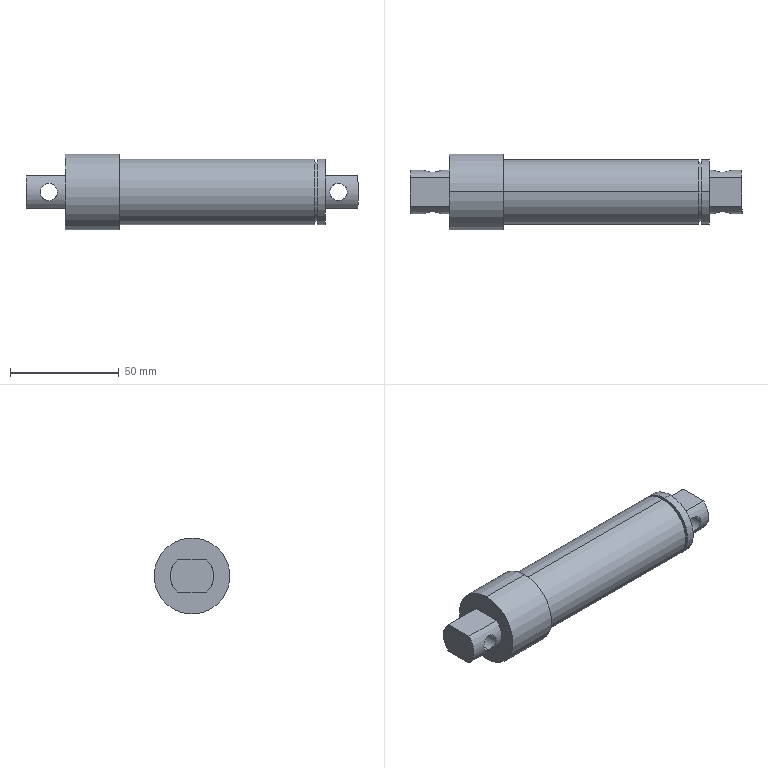Component | SolidWorks | LowerSideBeltXG-XG1-1_DrivenPulleyShaftXG-XG1-1 | 1 solid | 27 faces | box 153 x 35 x 35 mm | volume 97945 mm3 | cylinder 16 | plane 11 | commonest cylinder face diameters 8 x4 30 x4 20 x4 35 x2 27 x2
STEP:
#1=COLOUR_RGB('',0.7922,0.8196,0.9333);
#2=FILL_AREA_STYLE_COLOUR('',#1);
#3=FILL_AREA_STYLE('',(#2));
#4=SURFACE_STYLE_FILL_AREA(#3);
#5=SURFACE_SIDE_STYLE('',(#4));
#6=SURFACE_STYLE_USAGE(.BOTH.,#5);
#7=PRESENTATION_STYLE_ASSIGNMENT((#6));
#8=CARTESIAN_POINT('',(-7.489,10.853,4.331));
#9=VERTEX_POINT('',#8);
#10=CARTESIAN_POINT('',(-7.489,10.853,4.646));
#11=VERTEX_POINT('',#10);
#12=CARTESIAN_POINT('',(-7.489,10.853,4.331));
#13=CARTESIAN_POINT('',(-7.479,10.853,4.331));
#14=CARTESIAN_POINT('',(-7.468,10.853,4.332));
#15=CARTESIAN_POINT('',(-7.448,10.855,4.336));
#16=CARTESIAN_POINT('',(-7.438,10.856,4.339));
#17=CARTESIAN_POINT('',(-7.419,10.86,4.347));
#18=CARTESIAN_POINT('',(-7.41,10.861,4.352));
#19=CARTESIAN_POINT('',(-7.393,10.865,4.363));
#20=CARTESIAN_POINT('',(-7.385,10.868,4.37));
#21=CARTESIAN_POINT('',(-7.37,10.872,4.384));
#22=CARTESIAN_POINT('',(-7.364,10.874,4.392));
#23=CARTESIAN_POINT('',(-7.353,10.878,4.409));
#24=CARTESIAN_POINT('',(-7.348,10.88,4.418));
#25=CARTESIAN_POINT('',(-7.34,10.883,4.437));
#26=CARTESIAN_POINT('',(-7.337,10.884,4.447));
#27=CARTESIAN_POINT('',(-7.333,10.885,4.467));
#28=CARTESIAN_POINT('',(-7.331,10.886,4.478));
#29=CARTESIAN_POINT('',(-7.331,10.886,4.498));
#30=CARTESIAN_POINT('',(-7.332,10.885,4.509));
#31=CARTESIAN_POINT('',(-7.337,10.884,4.529));
#32=CARTESIAN_POINT('',(-7.34,10.883,4.539));
#33=CARTESIAN_POINT('',(-7.348,10.88,4.558));
#34=CARTESIAN_POINT('',(-7.352,10.878,4.567));
#35=CARTESIAN_POINT('',(-7.364,10.874,4.584));
#36=CARTESIAN_POINT('',(-7.37,10.872,4.592));
#37=CARTESIAN_POINT('',(-7.385,10.868,4.607));
#38=CARTESIAN_POINT('',(-7.393,10.865,4.613));
#39=CARTESIAN_POINT('',(-7.41,10.861,4.625));
#40=CARTESIAN_POINT('',(-7.419,10.86,4.629));
#41=CARTESIAN_POINT('',(-7.438,10.856,4.637));
#42=CARTESIAN_POINT('',(-7.448,10.855,4.641));
#43=CARTESIAN_POINT('',(-7.468,10.853,4.645));
#44=CARTESIAN_POINT('',(-7.478,10.853,4.646));
#45=CARTESIAN_POINT('',(-7.489,10.853,4.646));
#46=B_SPLINE_CURVE_WITH_KNOTS('',3,(#12,#13,#14,#15,#16,#17,#18,#19,#20,#21,#22,#23,#24,#25,#26,#27,#28,#29,#30,#31,#32,#33,#34,#35,#36,#37,#38,#39,#40,#41,#42,#43,#44,#45),.UNSPECIFIED.,.F.,.F.,(4,2,2,2,2,2,2,2,2,2,2,2,2,2,2,2,4),(0.01264,0.01343,0.01422,0.01501,0.0158,0.01658,0.01737,0.01816,0.01895,0.01974,0.02053,0.02132,0.02211,0.0229,0.02369,0.02448,0.02527),.UNSPECIFIED.);
#47=EDGE_CURVE('',#9,#11,#46,.T.);
#48=ORIENTED_EDGE('',*,*,#47,.F.);
#49=CARTESIAN_POINT('',(-7.489,10.131,4.331));
#50=VERTEX_POINT('',#49);
#51=CARTESIAN_POINT('',(-7.489,10.098,4.331));
#52=DIRECTION('',(0.,-1.,-0.));
#53=VECTOR('',#52,39.37);
#54=LINE('',#51,#53);
#55=EDGE_CURVE('',#9,#50,#54,.T.);
#56=ORIENTED_EDGE('',*,*,#55,.T.);
#57=CARTESIAN_POINT('',(-7.489,10.131,4.646));
#58=VERTEX_POINT('',#57);
#59=CARTESIAN_POINT('',(-7.489,10.131,4.646));
#60=CARTESIAN_POINT('',(-7.478,10.131,4.646));
#61=CARTESIAN_POINT('',(-7.468,10.131,4.645));
#62=CARTESIAN_POINT('',(-7.448,10.129,4.641));
#63=CARTESIAN_POINT('',(-7.438,10.128,4.637));
#64=CARTESIAN_POINT('',(-7.419,10.125,4.63));
#65=CARTESIAN_POINT('',(-7.41,10.123,4.625));
#66=CARTESIAN_POINT('',(-7.393,10.119,4.613));
#67=CARTESIAN_POINT('',(-7.385,10.117,4.607));
#68=CARTESIAN_POINT('',(-7.37,10.112,4.592));
#69=CARTESIAN_POINT('',(-7.364,10.11,4.584));
#70=CARTESIAN_POINT('',(-7.352,10.106,4.567));
#71=CARTESIAN_POINT('',(-7.348,10.105,4.558));
#72=CARTESIAN_POINT('',(-7.34,10.102,4.539));
#73=CARTESIAN_POINT('',(-7.337,10.1,4.529));
#74=CARTESIAN_POINT('',(-7.333,10.099,4.509));
#75=CARTESIAN_POINT('',(-7.331,10.098,4.499));
#76=CARTESIAN_POINT('',(-7.331,10.098,4.478));
#77=CARTESIAN_POINT('',(-7.333,10.099,4.467));
#78=CARTESIAN_POINT('',(-7.337,10.1,4.447));
#79=CARTESIAN_POINT('',(-7.34,10.102,4.437));
#80=CARTESIAN_POINT('',(-7.348,10.105,4.418));
#81=CARTESIAN_POINT('',(-7.353,10.106,4.409));
#82=CARTESIAN_POINT('',(-7.364,10.11,4.392));
#83=CARTESIAN_POINT('',(-7.371,10.112,4.384));
#84=CARTESIAN_POINT('',(-7.385,10.117,4.37));
#85=CARTESIAN_POINT('',(-7.393,10.119,4.363));
#86=CARTESIAN_POINT('',(-7.41,10.123,4.352));
#87=CARTESIAN_POINT('',(-7.419,10.125,4.347));
#88=CARTESIAN_POINT('',(-7.438,10.128,4.339));
#89=CARTESIAN_POINT('',(-7.448,10.129,4.336));
#90=CARTESIAN_POINT('',(-7.468,10.131,4.332));
#91=CARTESIAN_POINT('',(-7.479,10.131,4.331));
#92=CARTESIAN_POINT('',(-7.489,10.131,4.331));
#93=B_SPLINE_CURVE_WITH_KNOTS('',3,(#59,#60,#61,#62,#63,#64,#65,#66,#67,#68,#69,#70,#71,#72,#73,#74,#75,#76,#77,#78,#79,#80,#81,#82,#83,#84,#85,#86,#87,#88,#89,#90,#91,#92),.UNSPECIFIED.,.F.,.F.,(4,2,2,2,2,2,2,2,2,2,2,2,2,2,2,2,4),(0.,0.0007899,0.00158,0.00237,0.00316,0.00395,0.00474,0.00553,0.006319,0.007109,0.007899,0.008689,0.009479,0.01027,0.01106,0.01185,0.01264),.UNSPECIFIED.);
#94=EDGE_CURVE('',#58,#50,#93,.T.);
#95=ORIENTED_EDGE('',*,*,#94,.F.);
#96=CARTESIAN_POINT('',(-7.489,10.098,4.646));
#97=DIRECTION('',(0.,-1.,-0.));
#98=VECTOR('',#97,39.37);
#99=LINE('',#96,#98);
#100=EDGE_CURVE('',#11,#58,#99,.T.);
#101=ORIENTED_EDGE('',*,*,#100,.F.);
#102=EDGE_LOOP('',(#48,#56,#95,#101));
#103=FACE_OUTER_BOUND('',#102,.T.);
#104=CARTESIAN_POINT('',(-7.489,10.098,4.488));
#105=DIRECTION('',(0.,-1.,-0.));
#106=DIRECTION('',(0.,0.,1.));
#107=AXIS2_PLACEMENT_3D('',#104,#105,#106);
#108=CYLINDRICAL_SURFACE('',#107,0.1575);
#109=ADVANCED_FACE('',(#103),#108,.F.);
#110=CARTESIAN_POINT('',(-12.745,10.853,4.646));
#111=VERTEX_POINT('',#110);
#112=CARTESIAN_POINT('',(-12.745,10.853,4.331));
#113=VERTEX_POINT('',#112);
#114=CARTESIAN_POINT('',(-12.745,10.853,4.646));
#115=CARTESIAN_POINT('',(-12.734,10.853,4.646));
#116=CARTESIAN_POINT('',(-12.724,10.853,4.645));
#117=CARTESIAN_POINT('',(-12.704,10.855,4.641));
#118=CARTESIAN_POINT('',(-12.694,10.856,4.637));
#119=CARTESIAN_POINT('',(-12.675,10.86,4.63));
#120=CARTESIAN_POINT('',(-12.666,10.861,4.625));
#121=CARTESIAN_POINT('',(-12.649,10.865,4.613));
#122=CARTESIAN_POINT('',(-12.641,10.868,4.607));
#123=CARTESIAN_POINT('',(-12.626,10.872,4.592));
#124=CARTESIAN_POINT('',(-12.62,10.874,4.584));
#125=CARTESIAN_POINT('',(-12.608,10.878,4.567));
#126=CARTESIAN_POINT('',(-12.604,10.88,4.558));
#127=CARTESIAN_POINT('',(-12.596,10.883,4.539));
#128=CARTESIAN_POINT('',(-12.593,10.884,4.529));
#129=CARTESIAN_POINT('',(-12.588,10.885,4.509));
#130=CARTESIAN_POINT('',(-12.587,10.886,4.499));
#131=CARTESIAN_POINT('',(-12.587,10.886,4.478));
#132=CARTESIAN_POINT('',(-12.588,10.885,4.467));
#133=CARTESIAN_POINT('',(-12.593,10.884,4.447));
#134=CARTESIAN_POINT('',(-12.596,10.883,4.437));
#135=CARTESIAN_POINT('',(-12.604,10.88,4.418));
#136=CARTESIAN_POINT('',(-12.608,10.878,4.409));
#137=CARTESIAN_POINT('',(-12.62,10.874,4.392));
#138=CARTESIAN_POINT('',(-12.626,10.872,4.384));
#139=CARTESIAN_POINT('',(-12.641,10.868,4.37));
#140=CARTESIAN_POINT('',(-12.649,10.865,4.363));
#141=CARTESIAN_POINT('',(-12.666,10.861,4.352));
#142=CARTESIAN_POINT('',(-12.675,10.86,4.347));
#143=CARTESIAN_POINT('',(-12.694,10.856,4.339));
#144=CARTESIAN_POINT('',(-12.704,10.855,4.336));
#145=CARTESIAN_POINT('',(-12.724,10.853,4.332));
#146=CARTESIAN_POINT('',(-12.735,10.853,4.331));
#147=CARTESIAN_POINT('',(-12.745,10.853,4.331));
#148=B_SPLINE_CURVE_WITH_KNOTS('',3,(#114,#115,#116,#117,#118,#119,#120,#121,#122,#123,#124,#125,#126,#127,#128,#129,#130,#131,#132,#133,#134,#135,#136,#137,#138,#139,#140,#141,#142,#143,#144,#145,#146,#147),.UNSPECIFIED.,.F.,.F.,(4,2,2,2,2,2,2,2,2,2,2,2,2,2,2,2,4),(0.,0.0007899,0.00158,0.00237,0.00316,0.00395,0.00474,0.00553,0.006319,0.007109,0.007899,0.008689,0.009479,0.01027,0.01106,0.01185,0.01264),.UNSPECIFIED.);
#149=EDGE_CURVE('',#111,#113,#148,.T.);
#150=ORIENTED_EDGE('',*,*,#149,.T.);
#151=CARTESIAN_POINT('',(-12.745,10.131,4.331));
#152=VERTEX_POINT('',#151);
#153=CARTESIAN_POINT('',(-12.745,10.098,4.331));
#154=DIRECTION('',(0.,-1.,-0.));
#155=VECTOR('',#154,39.37);
#156=LINE('',#153,#155);
#157=EDGE_CURVE('',#113,#152,#156,.T.);
#158=ORIENTED_EDGE('',*,*,#157,.T.);
#159=CARTESIAN_POINT('',(-12.745,10.131,4.646));
#160=VERTEX_POINT('',#159);
#161=CARTESIAN_POINT('',(-12.745,10.131,4.331));
#162=CARTESIAN_POINT('',(-12.735,10.131,4.331));
#163=CARTESIAN_POINT('',(-12.724,10.131,4.332));
#164=CARTESIAN_POINT('',(-12.704,10.129,4.336));
#165=CARTESIAN_POINT('',(-12.694,10.128,4.339));
#166=CARTESIAN_POINT('',(-12.675,10.125,4.347));
#167=CARTESIAN_POINT('',(-12.666,10.123,4.352));
#168=CARTESIAN_POINT('',(-12.649,10.119,4.363));
#169=CARTESIAN_POINT('',(-12.641,10.117,4.37));
#170=CARTESIAN_POINT('',(-12.626,10.112,4.384));
#171=CARTESIAN_POINT('',(-12.62,10.11,4.392));
#172=CARTESIAN_POINT('',(-12.608,10.106,4.409));
#173=CARTESIAN_POINT('',(-12.604,10.105,4.418));
#174=CARTESIAN_POINT('',(-12.596,10.102,4.437));
#175=CARTESIAN_POINT('',(-12.593,10.1,4.447));
#176=CARTESIAN_POINT('',(-12.588,10.099,4.467));
#177=CARTESIAN_POINT('',(-12.587,10.098,4.478));
#178=CARTESIAN_POINT('',(-12.587,10.098,4.498));
#179=CARTESIAN_POINT('',(-12.588,10.099,4.509));
#180=CARTESIAN_POINT('',(-12.593,10.1,4.529));
#181=CARTESIAN_POINT('',(-12.596,10.102,4.539));
#182=CARTESIAN_POINT('',(-12.603,10.105,4.558));
#183=CARTESIAN_POINT('',(-12.608,10.106,4.567));
#184=CARTESIAN_POINT('',(-12.62,10.11,4.584));
#185=CARTESIAN_POINT('',(-12.626,10.112,4.592));
#186=CARTESIAN_POINT('',(-12.641,10.117,4.607));
#187=CARTESIAN_POINT('',(-12.649,10.119,4.613));
#188=CARTESIAN_POINT('',(-12.666,10.123,4.625));
#189=CARTESIAN_POINT('',(-12.675,10.125,4.629));
#190=CARTESIAN_POINT('',(-12.694,10.128,4.637));
#191=CARTESIAN_POINT('',(-12.704,10.129,4.641));
#192=CARTESIAN_POINT('',(-12.724,10.131,4.645));
#193=CARTESIAN_POINT('',(-12.734,10.131,4.646));
#194=CARTESIAN_POINT('',(-12.745,10.131,4.646));
#195=B_SPLINE_CURVE_WITH_KNOTS('',3,(#161,#162,#163,#164,#165,#166,#167,#168,#169,#170,#171,#172,#173,#174,#175,#176,#177,#178,#179,#180,#181,#182,#183,#184,#185,#186,#187,#188,#189,#190,#191,#192,#193,#194),.UNSPECIFIED.,.F.,.F.,(4,2,2,2,2,2,2,2,2,2,2,2,2,2,2,2,4),(0.01264,0.01343,0.01422,0.01501,0.0158,0.01658,0.01737,0.01816,0.01895,0.01974,0.02053,0.02132,0.02211,0.0229,0.02369,0.02448,0.02527),.UNSPECIFIED.);
#196=EDGE_CURVE('',#152,#160,#195,.T.);
#197=ORIENTED_EDGE('',*,*,#196,.T.);
#198=CARTESIAN_POINT('',(-12.745,10.098,4.646));
#199=DIRECTION('',(0.,-1.,-0.));
#200=VECTOR('',#199,39.37);
#201=LINE('',#198,#200);
#202=EDGE_CURVE('',#111,#160,#201,.T.);
#203=ORIENTED_EDGE('',*,*,#202,.F.);
#204=EDGE_LOOP('',(#150,#158,#197,#203));
#205=FACE_OUTER_BOUND('',#204,.T.);
#206=CARTESIAN_POINT('',(-12.745,10.098,4.488));
#207=DIRECTION('',(0.,-1.,-0.));
#208=DIRECTION('',(0.,0.,1.));
#209=AXIS2_PLACEMENT_3D('',#206,#207,#208);
#210=CYLINDRICAL_SURFACE('',#209,0.1575);
#211=ADVANCED_FACE('',(#205),#210,.F.);
#212=CARTESIAN_POINT('',(-12.45,10.492,3.799));
#213=VERTEX_POINT('',#212);
#214=CARTESIAN_POINT('',(-12.45,10.492,5.177));
#215=VERTEX_POINT('',#214);
#216=CARTESIAN_POINT('',(-12.45,10.492,4.488));
#217=DIRECTION('',(1.,0.,0.));
#218=DIRECTION('',(0.,0.,-1.));
#219=AXIS2_PLACEMENT_3D('',#216,#217,#218);
#220=CIRCLE('',#219,0.689);
#221=EDGE_CURVE('',#213,#215,#220,.T.);
#222=ORIENTED_EDGE('',*,*,#221,.T.);
#223=CARTESIAN_POINT('',(-11.465,10.492,5.177));
#224=VERTEX_POINT('',#223);
#225=CARTESIAN_POINT('',(13.589,10.492,5.177));
#226=DIRECTION('',(1.,0.,0.));
#227=VECTOR('',#226,39.37);
#228=LINE('',#225,#227);
#229=EDGE_CURVE('',#215,#224,#228,.T.);
#230=ORIENTED_EDGE('',*,*,#229,.T.);
#231=CARTESIAN_POINT('',(-11.465,10.492,3.799));
#232=VERTEX_POINT('',#231);
#233=CARTESIAN_POINT('',(-11.465,10.492,4.488));
#234=DIRECTION('',(1.,0.,0.));
#235=DIRECTION('',(0.,0.,-1.));
#236=AXIS2_PLACEMENT_3D('',#233,#234,#235);
#237=CIRCLE('',#236,0.689);
#238=EDGE_CURVE('',#232,#224,#237,.T.);
#239=ORIENTED_EDGE('',*,*,#238,.F.);
#240=CARTESIAN_POINT('',(13.589,10.492,3.799));
#241=DIRECTION('',(1.,0.,0.));
#242=VECTOR('',#241,39.37);
#243=LINE('',#240,#242);
#244=EDGE_CURVE('',#213,#232,#243,.T.);
#245=ORIENTED_EDGE('',*,*,#244,.F.);
#246=EDGE_LOOP('',(#222,#230,#239,#245));
#247=FACE_OUTER_BOUND('',#246,.T.);
#248=CARTESIAN_POINT('',(13.589,10.492,4.488));
#249=DIRECTION('',(1.,0.,0.));
#250=DIRECTION('',(0.,0.,-1.));
#251=AXIS2_PLACEMENT_3D('',#248,#249,#250);
#252=CYLINDRICAL_SURFACE('',#251,0.689);
#253=ADVANCED_FACE('',(#247),#252,.T.);
#254=CARTESIAN_POINT('',(-11.465,10.492,3.898));
#255=VERTEX_POINT('',#254);
#256=CARTESIAN_POINT('',(-11.465,10.492,5.079));
#257=VERTEX_POINT('',#256);
#258=CARTESIAN_POINT('',(-11.465,10.492,4.488));
#259=DIRECTION('',(1.,0.,0.));
#260=DIRECTION('',(0.,0.,-1.));
#261=AXIS2_PLACEMENT_3D('',#258,#259,#260);
#262=CIRCLE('',#261,0.5906);
#263=EDGE_CURVE('',#255,#257,#262,.T.);
#264=ORIENTED_EDGE('',*,*,#263,.T.);
#265=CARTESIAN_POINT('',(-7.922,10.492,5.079));
#266=VERTEX_POINT('',#265);
#267=CARTESIAN_POINT('',(13.589,10.492,5.079));
#268=DIRECTION('',(1.,0.,0.));
#269=VECTOR('',#268,39.37);
#270=LINE('',#267,#269);
#271=EDGE_CURVE('',#257,#266,#270,.T.);
#272=ORIENTED_EDGE('',*,*,#271,.T.);
#273=CARTESIAN_POINT('',(-7.922,10.492,3.898));
#274=VERTEX_POINT('',#273);
#275=CARTESIAN_POINT('',(-7.922,10.492,4.488));
#276=DIRECTION('',(1.,0.,0.));
#277=DIRECTION('',(0.,0.,-1.));
#278=AXIS2_PLACEMENT_3D('',#275,#276,#277);
#279=CIRCLE('',#278,0.5906);
#280=EDGE_CURVE('',#274,#266,#279,.T.);
#281=ORIENTED_EDGE('',*,*,#280,.F.);
#282=CARTESIAN_POINT('',(13.589,10.492,3.898));
#283=DIRECTION('',(1.,0.,0.));
#284=VECTOR('',#283,39.37);
#285=LINE('',#282,#284);
#286=EDGE_CURVE('',#255,#274,#285,.T.);
#287=ORIENTED_EDGE('',*,*,#286,.F.);
#288=EDGE_LOOP('',(#264,#272,#281,#287));
#289=FACE_OUTER_BOUND('',#288,.T.);
#290=CARTESIAN_POINT('',(13.589,10.492,4.488));
#291=DIRECTION('',(1.,0.,0.));
#292=DIRECTION('',(0.,0.,-1.));
#293=AXIS2_PLACEMENT_3D('',#290,#291,#292);
#294=CYLINDRICAL_SURFACE('',#293,0.5906);
#295=ADVANCED_FACE('',(#289),#294,.T.);
#296=CARTESIAN_POINT('',(-7.922,10.492,3.957));
#297=VERTEX_POINT('',#296);
#298=CARTESIAN_POINT('',(-7.922,10.492,5.02));
#299=VERTEX_POINT('',#298);
#300=CARTESIAN_POINT('',(-7.922,10.492,4.488));
#301=DIRECTION('',(1.,0.,0.));
#302=DIRECTION('',(0.,0.,-1.));
#303=AXIS2_PLACEMENT_3D('',#300,#301,#302);
#304=CIRCLE('',#303,0.5315);
#305=EDGE_CURVE('',#297,#299,#304,.T.);
#306=ORIENTED_EDGE('',*,*,#305,.T.);
#307=CARTESIAN_POINT('',(-7.875,10.492,5.02));
#308=VERTEX_POINT('',#307);
#309=CARTESIAN_POINT('',(13.589,10.492,5.02));
#310=DIRECTION('',(1.,0.,0.));
#311=VECTOR('',#310,39.37);
#312=LINE('',#309,#311);
#313=EDGE_CURVE('',#299,#308,#312,.T.);
#314=ORIENTED_EDGE('',*,*,#313,.T.);
#315=CARTESIAN_POINT('',(-7.875,10.492,3.957));
#316=VERTEX_POINT('',#315);
#317=CARTESIAN_POINT('',(-7.875,10.492,4.488));
#318=DIRECTION('',(1.,0.,0.));
#319=DIRECTION('',(0.,0.,-1.));
#320=AXIS2_PLACEMENT_3D('',#317,#318,#319);
#321=CIRCLE('',#320,0.5315);
#322=EDGE_CURVE('',#316,#308,#321,.T.);
#323=ORIENTED_EDGE('',*,*,#322,.F.);
#324=CARTESIAN_POINT('',(13.589,10.492,3.957));
#325=DIRECTION('',(1.,0.,0.));
#326=VECTOR('',#325,39.37);
#327=LINE('',#324,#326);
#328=EDGE_CURVE('',#297,#316,#327,.T.);
#329=ORIENTED_EDGE('',*,*,#328,.F.);
#330=EDGE_LOOP('',(#306,#314,#323,#329));
#331=FACE_OUTER_BOUND('',#330,.T.);
#332=CARTESIAN_POINT('',(13.589,10.492,4.488));
#333=DIRECTION('',(1.,0.,0.));
#334=DIRECTION('',(0.,0.,-1.));
#335=AXIS2_PLACEMENT_3D('',#332,#333,#334);
#336=CYLINDRICAL_SURFACE('',#335,0.5315);
#337=ADVANCED_FACE('',(#331),#336,.T.);
#338=CARTESIAN_POINT('',(-7.875,10.492,3.898));
#339=VERTEX_POINT('',#338);
#340=CARTESIAN_POINT('',(-7.875,10.492,5.079));
#341=VERTEX_POINT('',#340);
#342=CARTESIAN_POINT('',(-7.875,10.492,4.488));
#343=DIRECTION('',(1.,0.,0.));
#344=DIRECTION('',(0.,0.,-1.));
#345=AXIS2_PLACEMENT_3D('',#342,#343,#344);
#346=CIRCLE('',#345,0.5906);
#347=EDGE_CURVE('',#339,#341,#346,.T.);
#348=ORIENTED_EDGE('',*,*,#347,.T.);
#349=CARTESIAN_POINT('',(-7.725,10.492,5.079));
#350=VERTEX_POINT('',#349);
#351=CARTESIAN_POINT('',(13.589,10.492,5.079));
#352=DIRECTION('',(1.,0.,0.));
#353=VECTOR('',#352,39.37);
#354=LINE('',#351,#353);
#355=EDGE_CURVE('',#341,#350,#354,.T.);
#356=ORIENTED_EDGE('',*,*,#355,.T.);
#357=CARTESIAN_POINT('',(-7.725,10.492,3.898));
#358=VERTEX_POINT('',#357);
#359=CARTESIAN_POINT('',(-7.725,10.492,4.488));
#360=DIRECTION('',(1.,0.,0.));
#361=DIRECTION('',(0.,0.,-1.));
#362=AXIS2_PLACEMENT_3D('',#359,#360,#361);
#363=CIRCLE('',#362,0.5906);
#364=EDGE_CURVE('',#358,#350,#363,.T.);
#365=ORIENTED_EDGE('',*,*,#364,.F.);
#366=CARTESIAN_POINT('',(13.589,10.492,3.898));
#367=DIRECTION('',(1.,0.,0.));
#368=VECTOR('',#367,39.37);
#369=LINE('',#366,#368);
#370=EDGE_CURVE('',#339,#358,#369,.T.);
#371=ORIENTED_EDGE('',*,*,#370,.F.);
#372=EDGE_LOOP('',(#348,#356,#365,#371));
#373=FACE_OUTER_BOUND('',#372,.T.);
#374=CARTESIAN_POINT('',(13.589,10.492,4.488));
#375=DIRECTION('',(1.,0.,0.));
#376=DIRECTION('',(0.,0.,-1.));
#377=AXIS2_PLACEMENT_3D('',#374,#375,#376);
#378=CYLINDRICAL_SURFACE('',#377,0.5906);
#379=ADVANCED_FACE('',(#373),#378,.T.);
#380=CARTESIAN_POINT('',(-12.745,10.131,4.646));
#381=CARTESIAN_POINT('',(-12.755,10.131,4.646));
#382=CARTESIAN_POINT('',(-12.766,10.131,4.645));
#383=CARTESIAN_POINT('',(-12.786,10.129,4.641));
#384=CARTESIAN_POINT('',(-12.796,10.128,4.637));
#385=CARTESIAN_POINT('',(-12.815,10.125,4.63));
#386=CARTESIAN_POINT('',(-12.824,10.123,4.625));
#387=CARTESIAN_POINT('',(-12.841,10.119,4.613));
#388=CARTESIAN_POINT('',(-12.849,10.117,4.607));
#389=CARTESIAN_POINT('',(-12.863,10.112,4.592));
#390=CARTESIAN_POINT('',(-12.87,10.11,4.584));
#391=CARTESIAN_POINT('',(-12.881,10.106,4.567));
#392=CARTESIAN_POINT('',(-12.886,10.105,4.558));
#393=CARTESIAN_POINT('',(-12.894,10.102,4.539));
#394=CARTESIAN_POINT('',(-12.897,10.1,4.529));
#395=CARTESIAN_POINT('',(-12.901,10.099,4.509));
#396=CARTESIAN_POINT('',(-12.902,10.098,4.499));
#397=CARTESIAN_POINT('',(-12.902,10.098,4.478));
#398=CARTESIAN_POINT('',(-12.901,10.099,4.467));
#399=CARTESIAN_POINT('',(-12.897,10.1,4.447));
#400=CARTESIAN_POINT('',(-12.894,10.102,4.437));
#401=CARTESIAN_POINT('',(-12.886,10.105,4.418));
#402=CARTESIAN_POINT('',(-12.881,10.106,4.409));
#403=CARTESIAN_POINT('',(-12.87,10.11,4.392));
#404=CARTESIAN_POINT('',(-12.863,10.112,4.384));
#405=CARTESIAN_POINT('',(-12.849,10.117,4.37));
#406=CARTESIAN_POINT('',(-12.841,10.119,4.363));
#407=CARTESIAN_POINT('',(-12.824,10.123,4.352));
#408=CARTESIAN_POINT('',(-12.815,10.125,4.347));
#409=CARTESIAN_POINT('',(-12.796,10.128,4.339));
#410=CARTESIAN_POINT('',(-12.786,10.129,4.336));
#411=CARTESIAN_POINT('',(-12.766,10.131,4.332));
#412=CARTESIAN_POINT('',(-12.755,10.131,4.331));
#413=CARTESIAN_POINT('',(-12.745,10.131,4.331));
#414=B_SPLINE_CURVE_WITH_KNOTS('',3,(#380,#381,#382,#383,#384,#385,#386,#387,#388,#389,#390,#391,#392,#393,#394,#395,#396,#397,#398,#399,#400,#401,#402,#403,#404,#405,#406,#407,#408,#409,#410,#411,#412,#413),.UNSPECIFIED.,.F.,.F.,(4,2,2,2,2,2,2,2,2,2,2,2,2,2,2,2,4),(0.,0.0007899,0.00158,0.00237,0.00316,0.00395,0.00474,0.00553,0.006319,0.007109,0.007899,0.008689,0.009479,0.01027,0.01106,0.01185,0.01264),.UNSPECIFIED.);
#415=EDGE_CURVE('',#160,#152,#414,.T.);
#416=ORIENTED_EDGE('',*,*,#415,.F.);
#417=ORIENTED_EDGE('',*,*,#196,.F.);
#418=EDGE_LOOP('',(#416,#417));
#419=FACE_BOUND('',#418,.T.);
#420=CARTESIAN_POINT('',(-13.158,10.232,4.783));
#421=VERTEX_POINT('',#420);
#422=CARTESIAN_POINT('',(-12.45,10.232,4.783));
#423=VERTEX_POINT('',#422);
#424=CARTESIAN_POINT('',(-12.45,10.232,4.783));
#425=DIRECTION('',(1.,0.,0.));
#426=VECTOR('',#425,39.37);
#427=LINE('',#424,#426);
#428=EDGE_CURVE('',#421,#423,#427,.T.);
#429=ORIENTED_EDGE('',*,*,#428,.F.);
#430=CARTESIAN_POINT('',(-13.158,10.232,4.193));
#431=VERTEX_POINT('',#430);
#432=CARTESIAN_POINT('',(-13.158,10.492,4.488));
#433=DIRECTION('',(1.,0.,0.));
#434=DIRECTION('',(0.,0.,-1.));
#435=AXIS2_PLACEMENT_3D('',#432,#433,#434);
#436=CIRCLE('',#435,0.3937);
#437=EDGE_CURVE('',#421,#431,#436,.T.);
#438=ORIENTED_EDGE('',*,*,#437,.T.);
#439=CARTESIAN_POINT('',(-12.45,10.232,4.193));
#440=VERTEX_POINT('',#439);
#441=CARTESIAN_POINT('',(-12.45,10.232,4.193));
#442=DIRECTION('',(-1.,-0.,-0.));
#443=VECTOR('',#442,39.37);
#444=LINE('',#441,#443);
#445=EDGE_CURVE('',#440,#431,#444,.T.);
#446=ORIENTED_EDGE('',*,*,#445,.F.);
#447=CARTESIAN_POINT('',(-12.45,10.492,4.488));
#448=DIRECTION('',(-1.,-0.,-0.));
#449=DIRECTION('',(0.,0.,1.));
#450=AXIS2_PLACEMENT_3D('',#447,#448,#449);
#451=CIRCLE('',#450,0.3937);
#452=EDGE_CURVE('',#440,#423,#451,.T.);
#453=ORIENTED_EDGE('',*,*,#452,.T.);
#454=EDGE_LOOP('',(#429,#438,#446,#453));
#455=FACE_OUTER_BOUND('',#454,.T.);
#456=CARTESIAN_POINT('',(-12.45,10.492,4.488));
#457=DIRECTION('',(-1.,-0.,-0.));
#458=DIRECTION('',(0.,0.,1.));
#459=AXIS2_PLACEMENT_3D('',#456,#457,#458);
#460=CYLINDRICAL_SURFACE('',#459,0.3937);
#461=ADVANCED_FACE('',(#419,#455),#460,.T.);
#462=ORIENTED_EDGE('',*,*,#94,.T.);
#463=CARTESIAN_POINT('',(-7.489,10.131,4.331));
#464=CARTESIAN_POINT('',(-7.499,10.131,4.331));
#465=CARTESIAN_POINT('',(-7.51,10.131,4.332));
#466=CARTESIAN_POINT('',(-7.53,10.129,4.336));
#467=CARTESIAN_POINT('',(-7.54,10.128,4.339));
#468=CARTESIAN_POINT('',(-7.559,10.125,4.347));
#469=CARTESIAN_POINT('',(-7.568,10.123,4.352));
#470=CARTESIAN_POINT('',(-7.585,10.119,4.363));
#471=CARTESIAN_POINT('',(-7.593,10.117,4.37));
#472=CARTESIAN_POINT('',(-7.608,10.112,4.384));
#473=CARTESIAN_POINT('',(-7.614,10.11,4.392));
#474=CARTESIAN_POINT('',(-7.625,10.106,4.409));
#475=CARTESIAN_POINT('',(-7.63,10.105,4.418));
#476=CARTESIAN_POINT('',(-7.638,10.102,4.437));
#477=CARTESIAN_POINT('',(-7.641,10.1,4.447));
#478=CARTESIAN_POINT('',(-7.645,10.099,4.467));
#479=CARTESIAN_POINT('',(-7.646,10.098,4.478));
#480=CARTESIAN_POINT('',(-7.646,10.098,4.498));
#481=CARTESIAN_POINT('',(-7.645,10.099,4.509));
#482=CARTESIAN_POINT('',(-7.641,10.1,4.529));
#483=CARTESIAN_POINT('',(-7.638,10.102,4.539));
#484=CARTESIAN_POINT('',(-7.63,10.105,4.558));
#485=CARTESIAN_POINT('',(-7.625,10.106,4.567));
#486=CARTESIAN_POINT('',(-7.614,10.11,4.584));
#487=CARTESIAN_POINT('',(-7.608,10.112,4.592));
#488=CARTESIAN_POINT('',(-7.593,10.117,4.607));
#489=CARTESIAN_POINT('',(-7.585,10.119,4.613));
#490=CARTESIAN_POINT('',(-7.568,10.123,4.625));
#491=CARTESIAN_POINT('',(-7.559,10.125,4.629));
#492=CARTESIAN_POINT('',(-7.54,10.128,4.637));
#493=CARTESIAN_POINT('',(-7.53,10.129,4.641));
#494=CARTESIAN_POINT('',(-7.51,10.131,4.645));
#495=CARTESIAN_POINT('',(-7.499,10.131,4.646));
#496=CARTESIAN_POINT('',(-7.489,10.131,4.646));
#497=B_SPLINE_CURVE_WITH_KNOTS('',3,(#463,#464,#465,#466,#467,#468,#469,#470,#471,#472,#473,#474,#475,#476,#477,#478,#479,#480,#481,#482,#483,#484,#485,#486,#487,#488,#489,#490,#491,#492,#493,#494,#495,#496),.UNSPECIFIED.,.F.,.F.,(4,2,2,2,2,2,2,2,2,2,2,2,2,2,2,2,4),(0.01264,0.01343,0.01422,0.01501,0.0158,0.01658,0.01737,0.01816,0.01895,0.01974,0.02053,0.02132,0.02211,0.0229,0.02369,0.02448,0.02527),.UNSPECIFIED.);
#498=EDGE_CURVE('',#50,#58,#497,.T.);
#499=ORIENTED_EDGE('',*,*,#498,.T.);
#500=EDGE_LOOP('',(#462,#499));
#501=FACE_BOUND('',#500,.T.);
#502=CARTESIAN_POINT('',(-7.135,10.232,4.783));
#503=VERTEX_POINT('',#502);
#504=CARTESIAN_POINT('',(-7.135,10.232,4.193));
#505=VERTEX_POINT('',#504);
#506=CARTESIAN_POINT('',(-7.135,10.492,4.488));
#507=DIRECTION('',(1.,0.,0.));
#508=DIRECTION('',(0.,0.,-1.));
#509=AXIS2_PLACEMENT_3D('',#506,#507,#508);
#510=CIRCLE('',#509,0.3937);
#511=EDGE_CURVE('',#503,#505,#510,.T.);
#512=ORIENTED_EDGE('',*,*,#511,.F.);
#513=CARTESIAN_POINT('',(-7.725,10.232,4.783));
#514=VERTEX_POINT('',#513);
#515=CARTESIAN_POINT('',(13.589,10.232,4.783));
#516=DIRECTION('',(-1.,-0.,-0.));
#517=VECTOR('',#516,39.37);
#518=LINE('',#515,#517);
#519=EDGE_CURVE('',#503,#514,#518,.T.);
#520=ORIENTED_EDGE('',*,*,#519,.T.);
#521=CARTESIAN_POINT('',(-7.725,10.232,4.193));
#522=VERTEX_POINT('',#521);
#523=CARTESIAN_POINT('',(-7.725,10.492,4.488));
#524=DIRECTION('',(1.,0.,0.));
#525=DIRECTION('',(0.,0.,-1.));
#526=AXIS2_PLACEMENT_3D('',#523,#524,#525);
#527=CIRCLE('',#526,0.3937);
#528=EDGE_CURVE('',#514,#522,#527,.T.);
#529=ORIENTED_EDGE('',*,*,#528,.T.);
#530=CARTESIAN_POINT('',(13.589,10.232,4.193));
#531=DIRECTION('',(1.,0.,0.));
#532=VECTOR('',#531,39.37);
#533=LINE('',#530,#532);
#534=EDGE_CURVE('',#522,#505,#533,.T.);
#535=ORIENTED_EDGE('',*,*,#534,.T.);
#536=EDGE_LOOP('',(#512,#520,#529,#535));
#537=FACE_OUTER_BOUND('',#536,.T.);
#538=CARTESIAN_POINT('',(13.589,10.492,4.488));
#539=DIRECTION('',(1.,0.,0.));
#540=DIRECTION('',(0.,0.,-1.));
#541=AXIS2_PLACEMENT_3D('',#538,#539,#540);
#542=CYLINDRICAL_SURFACE('',#541,0.3937);
#543=ADVANCED_FACE('',(#501,#537),#542,.T.);
#544=CARTESIAN_POINT('',(-7.489,10.853,4.646));
#545=CARTESIAN_POINT('',(-7.499,10.853,4.646));
#546=CARTESIAN_POINT('',(-7.51,10.853,4.645));
#547=CARTESIAN_POINT('',(-7.53,10.855,4.641));
#548=CARTESIAN_POINT('',(-7.54,10.856,4.637));
#549=CARTESIAN_POINT('',(-7.559,10.86,4.63));
#550=CARTESIAN_POINT('',(-7.568,10.861,4.625));
#551=CARTESIAN_POINT('',(-7.585,10.865,4.613));
#552=CARTESIAN_POINT('',(-7.593,10.868,4.607));
#553=CARTESIAN_POINT('',(-7.608,10.872,4.592));
#554=CARTESIAN_POINT('',(-7.614,10.874,4.584));
#555=CARTESIAN_POINT('',(-7.626,10.878,4.567));
#556=CARTESIAN_POINT('',(-7.63,10.88,4.558));
#557=CARTESIAN_POINT('',(-7.638,10.883,4.539));
#558=CARTESIAN_POINT('',(-7.641,10.884,4.529));
#559=CARTESIAN_POINT('',(-7.645,10.885,4.509));
#560=CARTESIAN_POINT('',(-7.646,10.886,4.499));
#561=CARTESIAN_POINT('',(-7.646,10.886,4.478));
#562=CARTESIAN_POINT('',(-7.645,10.885,4.467));
#563=CARTESIAN_POINT('',(-7.641,10.884,4.447));
#564=CARTESIAN_POINT('',(-7.638,10.883,4.437));
#565=CARTESIAN_POINT('',(-7.63,10.88,4.418));
#566=CARTESIAN_POINT('',(-7.625,10.878,4.409));
#567=CARTESIAN_POINT('',(-7.614,10.874,4.392));
#568=CARTESIAN_POINT('',(-7.607,10.872,4.384));
#569=CARTESIAN_POINT('',(-7.593,10.868,4.37));
#570=CARTESIAN_POINT('',(-7.585,10.865,4.363));
#571=CARTESIAN_POINT('',(-7.568,10.861,4.352));
#572=CARTESIAN_POINT('',(-7.559,10.86,4.347));
#573=CARTESIAN_POINT('',(-7.54,10.856,4.339));
#574=CARTESIAN_POINT('',(-7.53,10.855,4.336));
#575=CARTESIAN_POINT('',(-7.51,10.853,4.332));
#576=CARTESIAN_POINT('',(-7.499,10.853,4.331));
#577=CARTESIAN_POINT('',(-7.489,10.853,4.331));
#578=B_SPLINE_CURVE_WITH_KNOTS('',3,(#544,#545,#546,#547,#548,#549,#550,#551,#552,#553,#554,#555,#556,#557,#558,#559,#560,#561,#562,#563,#564,#565,#566,#567,#568,#569,#570,#571,#572,#573,#574,#575,#576,#577),.UNSPECIFIED.,.F.,.F.,(4,2,2,2,2,2,2,2,2,2,2,2,2,2,2,2,4),(0.,0.0007899,0.00158,0.00237,0.00316,0.00395,0.00474,0.00553,0.006319,0.007109,0.007899,0.008689,0.009479,0.01027,0.01106,0.01185,0.01264),.UNSPECIFIED.);
#579=EDGE_CURVE('',#11,#9,#578,.T.);
#580=ORIENTED_EDGE('',*,*,#579,.T.);
#581=ORIENTED_EDGE('',*,*,#47,.T.);
#582=EDGE_LOOP('',(#580,#581));
#583=FACE_BOUND('',#582,.T.);
#584=CARTESIAN_POINT('',(-7.135,10.753,4.193));
#585=VERTEX_POINT('',#584);
#586=CARTESIAN_POINT('',(-7.135,10.753,4.783));
#587=VERTEX_POINT('',#586);
#588=CARTESIAN_POINT('',(-7.135,10.492,4.488));
#589=DIRECTION('',(1.,0.,0.));
#590=DIRECTION('',(0.,0.,-1.));
#591=AXIS2_PLACEMENT_3D('',#588,#589,#590);
#592=CIRCLE('',#591,0.3937);
#593=EDGE_CURVE('',#585,#587,#592,.T.);
#594=ORIENTED_EDGE('',*,*,#593,.F.);
#595=CARTESIAN_POINT('',(-7.725,10.753,4.193));
#596=VERTEX_POINT('',#595);
#597=CARTESIAN_POINT('',(13.589,10.753,4.193));
#598=DIRECTION('',(-1.,-0.,-0.));
#599=VECTOR('',#598,39.37);
#600=LINE('',#597,#599);
#601=EDGE_CURVE('',#585,#596,#600,.T.);
#602=ORIENTED_EDGE('',*,*,#601,.T.);
#603=CARTESIAN_POINT('',(-7.725,10.753,4.783));
#604=VERTEX_POINT('',#603);
#605=CARTESIAN_POINT('',(-7.725,10.492,4.488));
#606=DIRECTION('',(1.,0.,0.));
#607=DIRECTION('',(0.,0.,-1.));
#608=AXIS2_PLACEMENT_3D('',#605,#606,#607);
#609=CIRCLE('',#608,0.3937);
#610=EDGE_CURVE('',#596,#604,#609,.T.);
#611=ORIENTED_EDGE('',*,*,#610,.T.);
#612=CARTESIAN_POINT('',(13.589,10.753,4.783));
#613=DIRECTION('',(1.,0.,0.));
#614=VECTOR('',#613,39.37);
#615=LINE('',#612,#614);
#616=EDGE_CURVE('',#604,#587,#615,.T.);
#617=ORIENTED_EDGE('',*,*,#616,.T.);
#618=EDGE_LOOP('',(#594,#602,#611,#617));
#619=FACE_OUTER_BOUND('',#618,.T.);
#620=CARTESIAN_POINT('',(13.589,10.492,4.488));
#621=DIRECTION('',(1.,0.,0.));
#622=DIRECTION('',(0.,0.,-1.));
#623=AXIS2_PLACEMENT_3D('',#620,#621,#622);
#624=CYLINDRICAL_SURFACE('',#623,0.3937);
#625=ADVANCED_FACE('',(#583,#619),#624,.T.);
#626=CARTESIAN_POINT('',(-7.135,10.753,4.783));
#627=DIRECTION('',(0.,-1.,-0.));
#628=VECTOR('',#627,39.37);
#629=LINE('',#626,#628);
#630=EDGE_CURVE('',#587,#503,#629,.T.);
#631=ORIENTED_EDGE('',*,*,#630,.F.);
#632=ORIENTED_EDGE('',*,*,#616,.F.);
#633=CARTESIAN_POINT('',(-7.725,11.283,4.783));
#634=DIRECTION('',(-0.,1.,0.));
#635=VECTOR('',#634,39.37);
#636=LINE('',#633,#635);
#637=EDGE_CURVE('',#514,#604,#636,.T.);
#638=ORIENTED_EDGE('',*,*,#637,.F.);
#639=ORIENTED_EDGE('',*,*,#519,.F.);
#640=EDGE_LOOP('',(#631,#632,#638,#639));
#641=FACE_OUTER_BOUND('',#640,.T.);
#642=CARTESIAN_POINT('',(-7.725,11.283,4.783));
#643=DIRECTION('',(0.,0.,-1.));
#644=DIRECTION('',(0.,-1.,-0.));
#645=AXIS2_PLACEMENT_3D('',#642,#643,#644);
#646=PLANE('',#645);
#647=ADVANCED_FACE('',(#641),#646,.F.);
#648=CARTESIAN_POINT('',(-7.135,10.232,4.193));
#649=DIRECTION('',(-0.,1.,0.));
#650=VECTOR('',#649,39.37);
#651=LINE('',#648,#650);
#652=EDGE_CURVE('',#505,#585,#651,.T.);
#653=ORIENTED_EDGE('',*,*,#652,.F.);
#654=ORIENTED_EDGE('',*,*,#534,.F.);
#655=CARTESIAN_POINT('',(-7.725,11.283,4.193));
#656=DIRECTION('',(0.,-1.,-0.));
#657=VECTOR('',#656,39.37);
#658=LINE('',#655,#657);
#659=EDGE_CURVE('',#596,#522,#658,.T.);
#660=ORIENTED_EDGE('',*,*,#659,.F.);
#661=ORIENTED_EDGE('',*,*,#601,.F.);
#662=EDGE_LOOP('',(#653,#654,#660,#661));
#663=FACE_OUTER_BOUND('',#662,.T.);
#664=CARTESIAN_POINT('',(-7.725,11.283,4.193));
#665=DIRECTION('',(-0.,-0.,1.));
#666=DIRECTION('',(-0.,1.,0.));
#667=AXIS2_PLACEMENT_3D('',#664,#665,#666);
#668=PLANE('',#667);
#669=ADVANCED_FACE('',(#663),#668,.F.);
#670=ORIENTED_EDGE('',*,*,#610,.F.);
#671=ORIENTED_EDGE('',*,*,#659,.T.);
#672=ORIENTED_EDGE('',*,*,#528,.F.);
#673=ORIENTED_EDGE('',*,*,#637,.T.);
#674=EDGE_LOOP('',(#670,#671,#672,#673));
#675=FACE_BOUND('',#674,.T.);
#676=ORIENTED_EDGE('',*,*,#364,.T.);
#677=CARTESIAN_POINT('',(-7.725,10.492,4.488));
#678=DIRECTION('',(1.,0.,0.));
#679=DIRECTION('',(0.,0.,-1.));
#680=AXIS2_PLACEMENT_3D('',#677,#678,#679);
#681=CIRCLE('',#680,0.5906);
#682=EDGE_CURVE('',#350,#358,#681,.T.);
#683=ORIENTED_EDGE('',*,*,#682,.T.);
#684=EDGE_LOOP('',(#676,#683));
#685=FACE_OUTER_BOUND('',#684,.T.);
#686=CARTESIAN_POINT('',(-7.725,10.492,4.882));
#687=DIRECTION('',(-1.,-0.,-0.));
#688=DIRECTION('',(-0.,-0.,1.));
#689=AXIS2_PLACEMENT_3D('',#686,#687,#688);
#690=PLANE('',#689);
#691=ADVANCED_FACE('',(#675,#685),#690,.F.);
#692=ORIENTED_EDGE('',*,*,#355,.F.);
#693=CARTESIAN_POINT('',(-7.875,10.492,4.488));
#694=DIRECTION('',(1.,0.,0.));
#695=DIRECTION('',(0.,0.,-1.));
#696=AXIS2_PLACEMENT_3D('',#693,#694,#695);
#697=CIRCLE('',#696,0.5906);
#698=EDGE_CURVE('',#341,#339,#697,.T.);
#699=ORIENTED_EDGE('',*,*,#698,.T.);
#700=ORIENTED_EDGE('',*,*,#370,.T.);
#701=ORIENTED_EDGE('',*,*,#682,.F.);
#702=EDGE_LOOP('',(#692,#699,#700,#701));
#703=FACE_OUTER_BOUND('',#702,.T.);
#704=CARTESIAN_POINT('',(13.589,10.492,4.488));
#705=DIRECTION('',(1.,0.,0.));
#706=DIRECTION('',(0.,0.,-1.));
#707=AXIS2_PLACEMENT_3D('',#704,#705,#706);
#708=CYLINDRICAL_SURFACE('',#707,0.5906);
#709=ADVANCED_FACE('',(#703),#708,.T.);
#710=ORIENTED_EDGE('',*,*,#347,.F.);
#711=ORIENTED_EDGE('',*,*,#698,.F.);
#712=EDGE_LOOP('',(#710,#711));
#713=FACE_OUTER_BOUND('',#712,.T.);
#714=ORIENTED_EDGE('',*,*,#322,.T.);
#715=CARTESIAN_POINT('',(-7.875,10.492,4.488));
#716=DIRECTION('',(1.,0.,0.));
#717=DIRECTION('',(0.,0.,-1.));
#718=AXIS2_PLACEMENT_3D('',#715,#716,#717);
#719=CIRCLE('',#718,0.5315);
#720=EDGE_CURVE('',#308,#316,#719,.T.);
#721=ORIENTED_EDGE('',*,*,#720,.T.);
#722=EDGE_LOOP('',(#714,#721));
#723=FACE_BOUND('',#722,.T.);
#724=CARTESIAN_POINT('',(-7.875,10.492,5.079));
#725=DIRECTION('',(1.,0.,0.));
#726=DIRECTION('',(0.,0.,-1.));
#727=AXIS2_PLACEMENT_3D('',#724,#725,#726);
#728=PLANE('',#727);
#729=ADVANCED_FACE('',(#713,#723),#728,.F.);
#730=ORIENTED_EDGE('',*,*,#313,.F.);
#731=CARTESIAN_POINT('',(-7.922,10.492,4.488));
#732=DIRECTION('',(1.,0.,0.));
#733=DIRECTION('',(0.,0.,-1.));
#734=AXIS2_PLACEMENT_3D('',#731,#732,#733);
#735=CIRCLE('',#734,0.5315);
#736=EDGE_CURVE('',#299,#297,#735,.T.);
#737=ORIENTED_EDGE('',*,*,#736,.T.);
#738=ORIENTED_EDGE('',*,*,#328,.T.);
#739=ORIENTED_EDGE('',*,*,#720,.F.);
#740=EDGE_LOOP('',(#730,#737,#738,#739));
#741=FACE_OUTER_BOUND('',#740,.T.);
#742=CARTESIAN_POINT('',(13.589,10.492,4.488));
#743=DIRECTION('',(1.,0.,0.));
#744=DIRECTION('',(0.,0.,-1.));
#745=AXIS2_PLACEMENT_3D('',#742,#743,#744);
#746=CYLINDRICAL_SURFACE('',#745,0.5315);
#747=ADVANCED_FACE('',(#741),#746,.T.);
#748=ORIENTED_EDGE('',*,*,#305,.F.);
#749=ORIENTED_EDGE('',*,*,#736,.F.);
#750=EDGE_LOOP('',(#748,#749));
#751=FACE_BOUND('',#750,.T.);
#752=ORIENTED_EDGE('',*,*,#280,.T.);
#753=CARTESIAN_POINT('',(-7.922,10.492,4.488));
#754=DIRECTION('',(1.,0.,0.));
#755=DIRECTION('',(0.,0.,-1.));
#756=AXIS2_PLACEMENT_3D('',#753,#754,#755);
#757=CIRCLE('',#756,0.5906);
#758=EDGE_CURVE('',#266,#274,#757,.T.);
#759=ORIENTED_EDGE('',*,*,#758,.T.);
#760=EDGE_LOOP('',(#752,#759));
#761=FACE_OUTER_BOUND('',#760,.T.);
#762=CARTESIAN_POINT('',(-7.922,10.492,5.02));
#763=DIRECTION('',(-1.,-0.,-0.));
#764=DIRECTION('',(-0.,-0.,1.));
#765=AXIS2_PLACEMENT_3D('',#762,#763,#764);
#766=PLANE('',#765);
#767=ADVANCED_FACE('',(#751,#761),#766,.F.);
#768=ORIENTED_EDGE('',*,*,#271,.F.);
#769=CARTESIAN_POINT('',(-11.465,10.492,4.488));
#770=DIRECTION('',(1.,0.,0.));
#771=DIRECTION('',(0.,0.,-1.));
#772=AXIS2_PLACEMENT_3D('',#769,#770,#771);
#773=CIRCLE('',#772,0.5906);
#774=EDGE_CURVE('',#257,#255,#773,.T.);
#775=ORIENTED_EDGE('',*,*,#774,.T.);
#776=ORIENTED_EDGE('',*,*,#286,.T.);
#777=ORIENTED_EDGE('',*,*,#758,.F.);
#778=EDGE_LOOP('',(#768,#775,#776,#777));
#779=FACE_OUTER_BOUND('',#778,.T.);
#780=CARTESIAN_POINT('',(13.589,10.492,4.488));
#781=DIRECTION('',(1.,0.,0.));
#782=DIRECTION('',(0.,0.,-1.));
#783=AXIS2_PLACEMENT_3D('',#780,#781,#782);
#784=CYLINDRICAL_SURFACE('',#783,0.5906);
#785=ADVANCED_FACE('',(#779),#784,.T.);
#786=ORIENTED_EDGE('',*,*,#263,.F.);
#787=ORIENTED_EDGE('',*,*,#774,.F.);
#788=EDGE_LOOP('',(#786,#787));
#789=FACE_BOUND('',#788,.T.);
#790=ORIENTED_EDGE('',*,*,#238,.T.);
#791=CARTESIAN_POINT('',(-11.465,10.492,4.488));
#792=DIRECTION('',(1.,0.,0.));
#793=DIRECTION('',(0.,0.,-1.));
#794=AXIS2_PLACEMENT_3D('',#791,#792,#793);
#795=CIRCLE('',#794,0.689);
#796=EDGE_CURVE('',#224,#232,#795,.T.);
#797=ORIENTED_EDGE('',*,*,#796,.T.);
#798=EDGE_LOOP('',(#790,#797));
#799=FACE_OUTER_BOUND('',#798,.T.);
#800=CARTESIAN_POINT('',(-11.465,10.492,5.079));
#801=DIRECTION('',(-1.,-0.,-0.));
#802=DIRECTION('',(-0.,-0.,1.));
#803=AXIS2_PLACEMENT_3D('',#800,#801,#802);
#804=PLANE('',#803);
#805=ADVANCED_FACE('',(#789,#799),#804,.F.);
#806=ORIENTED_EDGE('',*,*,#229,.F.);
#807=CARTESIAN_POINT('',(-12.45,10.492,4.488));
#808=DIRECTION('',(1.,0.,0.));
#809=DIRECTION('',(0.,0.,-1.));
#810=AXIS2_PLACEMENT_3D('',#807,#808,#809);
#811=CIRCLE('',#810,0.689);
#812=EDGE_CURVE('',#215,#213,#811,.T.);
#813=ORIENTED_EDGE('',*,*,#812,.T.);
#814=ORIENTED_EDGE('',*,*,#244,.T.);
#815=ORIENTED_EDGE('',*,*,#796,.F.);
#816=EDGE_LOOP('',(#806,#813,#814,#815));
#817=FACE_OUTER_BOUND('',#816,.T.);
#818=CARTESIAN_POINT('',(13.589,10.492,4.488));
#819=DIRECTION('',(1.,0.,0.));
#820=DIRECTION('',(0.,0.,-1.));
#821=AXIS2_PLACEMENT_3D('',#818,#819,#820);
#822=CYLINDRICAL_SURFACE('',#821,0.689);
#823=ADVANCED_FACE('',(#817),#822,.T.);
#824=CARTESIAN_POINT('',(-12.45,10.753,4.783));
#825=VERTEX_POINT('',#824);
#826=CARTESIAN_POINT('',(-12.45,11.313,4.783));
#827=DIRECTION('',(0.,-1.,-0.));
#828=VECTOR('',#827,39.37);
#829=LINE('',#826,#828);
#830=EDGE_CURVE('',#825,#423,#829,.T.);
#831=ORIENTED_EDGE('',*,*,#830,.T.);
#832=ORIENTED_EDGE('',*,*,#452,.F.);
#833=CARTESIAN_POINT('',(-12.45,10.753,4.193));
#834=VERTEX_POINT('',#833);
#835=CARTESIAN_POINT('',(-12.45,11.313,4.193));
#836=DIRECTION('',(-0.,1.,0.));
#837=VECTOR('',#836,39.37);
#838=LINE('',#835,#837);
#839=EDGE_CURVE('',#440,#834,#838,.T.);
#840=ORIENTED_EDGE('',*,*,#839,.T.);
#841=CARTESIAN_POINT('',(-12.45,10.492,4.488));
#842=DIRECTION('',(-1.,-0.,-0.));
#843=DIRECTION('',(0.,0.,1.));
#844=AXIS2_PLACEMENT_3D('',#841,#842,#843);
#845=CIRCLE('',#844,0.3937);
#846=EDGE_CURVE('',#825,#834,#845,.T.);
#847=ORIENTED_EDGE('',*,*,#846,.F.);
#848=EDGE_LOOP('',(#831,#832,#840,#847));
#849=FACE_BOUND('',#848,.T.);
#850=ORIENTED_EDGE('',*,*,#221,.F.);
#851=ORIENTED_EDGE('',*,*,#812,.F.);
#852=EDGE_LOOP('',(#850,#851));
#853=FACE_OUTER_BOUND('',#852,.T.);
#854=CARTESIAN_POINT('',(-12.45,10.492,5.177));
#855=DIRECTION('',(1.,0.,0.));
#856=DIRECTION('',(0.,0.,-1.));
#857=AXIS2_PLACEMENT_3D('',#854,#855,#856);
#858=PLANE('',#857);
#859=ADVANCED_FACE('',(#849,#853),#858,.F.);
#860=ORIENTED_EDGE('',*,*,#511,.T.);
#861=ORIENTED_EDGE('',*,*,#652,.T.);
#862=ORIENTED_EDGE('',*,*,#593,.T.);
#863=ORIENTED_EDGE('',*,*,#630,.T.);
#864=EDGE_LOOP('',(#860,#861,#862,#863));
#865=FACE_OUTER_BOUND('',#864,.T.);
#866=CARTESIAN_POINT('',(-7.135,10.492,4.488));
#867=DIRECTION('',(1.,0.,0.));
#868=DIRECTION('',(0.,0.,-1.));
#869=AXIS2_PLACEMENT_3D('',#866,#867,#868);
#870=PLANE('',#869);
#871=ADVANCED_FACE('',(#865),#870,.T.);
#872=ORIENTED_EDGE('',*,*,#149,.F.);
#873=CARTESIAN_POINT('',(-12.745,10.853,4.331));
#874=CARTESIAN_POINT('',(-12.755,10.853,4.331));
#875=CARTESIAN_POINT('',(-12.766,10.853,4.332));
#876=CARTESIAN_POINT('',(-12.786,10.855,4.336));
#877=CARTESIAN_POINT('',(-12.796,10.856,4.339));
#878=CARTESIAN_POINT('',(-12.815,10.86,4.347));
#879=CARTESIAN_POINT('',(-12.824,10.861,4.352));
#880=CARTESIAN_POINT('',(-12.841,10.865,4.363));
#881=CARTESIAN_POINT('',(-12.849,10.868,4.37));
#882=CARTESIAN_POINT('',(-12.863,10.872,4.384));
#883=CARTESIAN_POINT('',(-12.87,10.874,4.392));
#884=CARTESIAN_POINT('',(-12.881,10.878,4.409));
#885=CARTESIAN_POINT('',(-12.886,10.88,4.418));
#886=CARTESIAN_POINT('',(-12.894,10.883,4.437));
#887=CARTESIAN_POINT('',(-12.897,10.884,4.447));
#888=CARTESIAN_POINT('',(-12.901,10.885,4.467));
#889=CARTESIAN_POINT('',(-12.902,10.886,4.478));
#890=CARTESIAN_POINT('',(-12.902,10.886,4.498));
#891=CARTESIAN_POINT('',(-12.901,10.885,4.509));
#892=CARTESIAN_POINT('',(-12.897,10.884,4.529));
#893=CARTESIAN_POINT('',(-12.894,10.883,4.539));
#894=CARTESIAN_POINT('',(-12.886,10.88,4.558));
#895=CARTESIAN_POINT('',(-12.881,10.878,4.567));
#896=CARTESIAN_POINT('',(-12.87,10.874,4.584));
#897=CARTESIAN_POINT('',(-12.863,10.872,4.592));
#898=CARTESIAN_POINT('',(-12.849,10.868,4.607));
#899=CARTESIAN_POINT('',(-12.841,10.865,4.613));
#900=CARTESIAN_POINT('',(-12.824,10.861,4.625));
#901=CARTESIAN_POINT('',(-12.815,10.86,4.629));
#902=CARTESIAN_POINT('',(-12.796,10.856,4.637));
#903=CARTESIAN_POINT('',(-12.786,10.855,4.641));
#904=CARTESIAN_POINT('',(-12.766,10.853,4.645));
#905=CARTESIAN_POINT('',(-12.755,10.853,4.646));
#906=CARTESIAN_POINT('',(-12.745,10.853,4.646));
#907=B_SPLINE_CURVE_WITH_KNOTS('',3,(#873,#874,#875,#876,#877,#878,#879,#880,#881,#882,#883,#884,#885,#886,#887,#888,#889,#890,#891,#892,#893,#894,#895,#896,#897,#898,#899,#900,#901,#902,#903,#904,#905,#906),.UNSPECIFIED.,.F.,.F.,(4,2,2,2,2,2,2,2,2,2,2,2,2,2,2,2,4),(0.01264,0.01343,0.01422,0.01501,0.0158,0.01658,0.01737,0.01816,0.01895,0.01974,0.02053,0.02132,0.02211,0.0229,0.02369,0.02448,0.02527),.UNSPECIFIED.);
#908=EDGE_CURVE('',#113,#111,#907,.T.);
#909=ORIENTED_EDGE('',*,*,#908,.F.);
#910=EDGE_LOOP('',(#872,#909));
#911=FACE_BOUND('',#910,.T.);
#912=CARTESIAN_POINT('',(-13.158,10.753,4.783));
#913=VERTEX_POINT('',#912);
#914=CARTESIAN_POINT('',(-12.45,10.753,4.783));
#915=DIRECTION('',(-1.,-0.,-0.));
#916=VECTOR('',#915,39.37);
#917=LINE('',#914,#916);
#918=EDGE_CURVE('',#825,#913,#917,.T.);
#919=ORIENTED_EDGE('',*,*,#918,.F.);
#920=ORIENTED_EDGE('',*,*,#846,.T.);
#921=CARTESIAN_POINT('',(-13.158,10.753,4.193));
#922=VERTEX_POINT('',#921);
#923=CARTESIAN_POINT('',(-12.45,10.753,4.193));
#924=DIRECTION('',(1.,0.,0.));
#925=VECTOR('',#924,39.37);
#926=LINE('',#923,#925);
#927=EDGE_CURVE('',#922,#834,#926,.T.);
#928=ORIENTED_EDGE('',*,*,#927,.F.);
#929=CARTESIAN_POINT('',(-13.158,10.492,4.488));
#930=DIRECTION('',(1.,0.,0.));
#931=DIRECTION('',(0.,0.,-1.));
#932=AXIS2_PLACEMENT_3D('',#929,#930,#931);
#933=CIRCLE('',#932,0.3937);
#934=EDGE_CURVE('',#922,#913,#933,.T.);
#935=ORIENTED_EDGE('',*,*,#934,.T.);
#936=EDGE_LOOP('',(#919,#920,#928,#935));
#937=FACE_OUTER_BOUND('',#936,.T.);
#938=CARTESIAN_POINT('',(-12.45,10.492,4.488));
#939=DIRECTION('',(-1.,-0.,-0.));
#940=DIRECTION('',(0.,0.,1.));
#941=AXIS2_PLACEMENT_3D('',#938,#939,#940);
#942=CYLINDRICAL_SURFACE('',#941,0.3937);
#943=ADVANCED_FACE('',(#911,#937),#942,.T.);
#944=ORIENTED_EDGE('',*,*,#437,.F.);
#945=CARTESIAN_POINT('',(-13.158,11.676,4.783));
#946=DIRECTION('',(-0.,1.,0.));
#947=VECTOR('',#946,39.37);
#948=LINE('',#945,#947);
#949=EDGE_CURVE('',#421,#913,#948,.T.);
#950=ORIENTED_EDGE('',*,*,#949,.T.);
#951=ORIENTED_EDGE('',*,*,#934,.F.);
#952=CARTESIAN_POINT('',(-13.158,11.676,4.193));
#953=DIRECTION('',(0.,-1.,-0.));
#954=VECTOR('',#953,39.37);
#955=LINE('',#952,#954);
#956=EDGE_CURVE('',#922,#431,#955,.T.);
#957=ORIENTED_EDGE('',*,*,#956,.T.);
#958=EDGE_LOOP('',(#944,#950,#951,#957));
#959=FACE_OUTER_BOUND('',#958,.T.);
#960=CARTESIAN_POINT('',(-13.158,11.676,3.799));
#961=DIRECTION('',(1.,0.,0.));
#962=DIRECTION('',(0.,0.,-1.));
#963=AXIS2_PLACEMENT_3D('',#960,#961,#962);
#964=PLANE('',#963);
#965=ADVANCED_FACE('',(#959),#964,.F.);
#966=ORIENTED_EDGE('',*,*,#927,.T.);
#967=ORIENTED_EDGE('',*,*,#839,.F.);
#968=ORIENTED_EDGE('',*,*,#445,.T.);
#969=ORIENTED_EDGE('',*,*,#956,.F.);
#970=EDGE_LOOP('',(#966,#967,#968,#969));
#971=FACE_OUTER_BOUND('',#970,.T.);
#972=CARTESIAN_POINT('',(-12.45,11.313,4.193));
#973=DIRECTION('',(-0.,-0.,1.));
#974=DIRECTION('',(-0.,1.,0.));
#975=AXIS2_PLACEMENT_3D('',#972,#973,#974);
#976=PLANE('',#975);
#977=ADVANCED_FACE('',(#971),#976,.F.);
#978=ORIENTED_EDGE('',*,*,#428,.T.);
#979=ORIENTED_EDGE('',*,*,#830,.F.);
#980=ORIENTED_EDGE('',*,*,#918,.T.);
#981=ORIENTED_EDGE('',*,*,#949,.F.);
#982=EDGE_LOOP('',(#978,#979,#980,#981));
#983=FACE_OUTER_BOUND('',#982,.T.);
#984=CARTESIAN_POINT('',(-12.45,11.313,4.783));
#985=DIRECTION('',(0.,0.,-1.));
#986=DIRECTION('',(0.,-1.,-0.));
#987=AXIS2_PLACEMENT_3D('',#984,#985,#986);
#988=PLANE('',#987);
#989=ADVANCED_FACE('',(#983),#988,.F.);
#990=ORIENTED_EDGE('',*,*,#157,.F.);
#991=ORIENTED_EDGE('',*,*,#908,.T.);
#992=ORIENTED_EDGE('',*,*,#202,.T.);
#993=ORIENTED_EDGE('',*,*,#415,.T.);
#994=EDGE_LOOP('',(#990,#991,#992,#993));
#995=FACE_OUTER_BOUND('',#994,.T.);
#996=CARTESIAN_POINT('',(-12.745,10.098,4.488));
#997=DIRECTION('',(0.,-1.,-0.));
#998=DIRECTION('',(0.,0.,1.));
#999=AXIS2_PLACEMENT_3D('',#996,#997,#998);
#1000=CYLINDRICAL_SURFACE('',#999,0.1575);
#1001=ADVANCED_FACE('',(#995),#1000,.F.);
#1002=ORIENTED_EDGE('',*,*,#55,.F.);
#1003=ORIENTED_EDGE('',*,*,#579,.F.);
#1004=ORIENTED_EDGE('',*,*,#100,.T.);
#1005=ORIENTED_EDGE('',*,*,#498,.F.);
#1006=EDGE_LOOP('',(#1002,#1003,#1004,#1005));
#1007=FACE_OUTER_BOUND('',#1006,.T.);
#1008=CARTESIAN_POINT('',(-7.489,10.098,4.488));
#1009=DIRECTION('',(0.,-1.,-0.));
#1010=DIRECTION('',(0.,0.,1.));
#1011=AXIS2_PLACEMENT_3D('',#1008,#1009,#1010);
#1012=CYLINDRICAL_SURFACE('',#1011,0.1575);
#1013=ADVANCED_FACE('',(#1007),#1012,.F.);
#1014=CLOSED_SHELL('',(#109,#211,#253,#295,#337,#379,#461,#543,#625,#647,#669,#691,#709,#729,#747,#767,#785,#805,#823,#859,#871,#943,#965,#977,#989,#1001,#1013));
#1015=MANIFOLD_SOLID_BREP('',#1014);
#1016=STYLED_ITEM('',(#7),#1015);
#1017=(LENGTH_UNIT()NAMED_UNIT(*)SI_UNIT($,.METRE.));
#1018=LENGTH_MEASURE_WITH_UNIT(LENGTH_MEASURE(0.0254),#1017);
#1019=DIMENSIONAL_EXPONENTS(1.,0.,0.,0.,0.,0.,0.);
#1020=(CONVERSION_BASED_UNIT('',#1018)LENGTH_UNIT()NAMED_UNIT(#1019));
#1021=UNCERTAINTY_MEASURE_WITH_UNIT(LENGTH_MEASURE(0.00001),#1020,'','');
#1022=(NAMED_UNIT(*)PLANE_ANGLE_UNIT()SI_UNIT($,.RADIAN.));
#1023=(NAMED_UNIT(*)SI_UNIT($,.STERADIAN.)SOLID_ANGLE_UNIT());
#1024=(GEOMETRIC_REPRESENTATION_CONTEXT(3)GLOBAL_UNCERTAINTY_ASSIGNED_CONTEXT((#1021))GLOBAL_UNIT_ASSIGNED_CONTEXT((#1020,#1022,#1023))REPRESENTATION_CONTEXT('',''));
#1025=MECHANICAL_DESIGN_GEOMETRIC_PRESENTATION_REPRESENTATION('',(#1016),#1024);
#1026=CARTESIAN_POINT('',(0.,0.,0.));
#1027=DIRECTION('',(0.,0.,1.));
#1028=DIRECTION('',(1.,0.,0.));
#1029=AXIS2_PLACEMENT_3D('',#1026,#1027,#1028);
#1030=(LENGTH_UNIT()NAMED_UNIT(*)SI_UNIT($,.METRE.));
#1031=LENGTH_MEASURE_WITH_UNIT(LENGTH_MEASURE(0.0254),#1030);
#1032=DIMENSIONAL_EXPONENTS(1.,0.,0.,0.,0.,0.,0.);
#1033=(CONVERSION_BASED_UNIT('',#1031)LENGTH_UNIT()NAMED_UNIT(#1032));
#1034=UNCERTAINTY_MEASURE_WITH_UNIT(LENGTH_MEASURE(0.00001),#1033,'','');
#1035=(NAMED_UNIT(*)PLANE_ANGLE_UNIT()SI_UNIT($,.RADIAN.));
#1036=(NAMED_UNIT(*)SI_UNIT($,.STERADIAN.)SOLID_ANGLE_UNIT());
#1037=(GEOMETRIC_REPRESENTATION_CONTEXT(3)GLOBAL_UNCERTAINTY_ASSIGNED_CONTEXT((#1034))GLOBAL_UNIT_ASSIGNED_CONTEXT((#1033,#1035,#1036))REPRESENTATION_CONTEXT('',''));
#1038=ADVANCED_BREP_SHAPE_REPRESENTATION('',(#1015,#1029),#1037);
#1039=PRESENTATION_LAYER_ASSIGNMENT('','',(#1016));